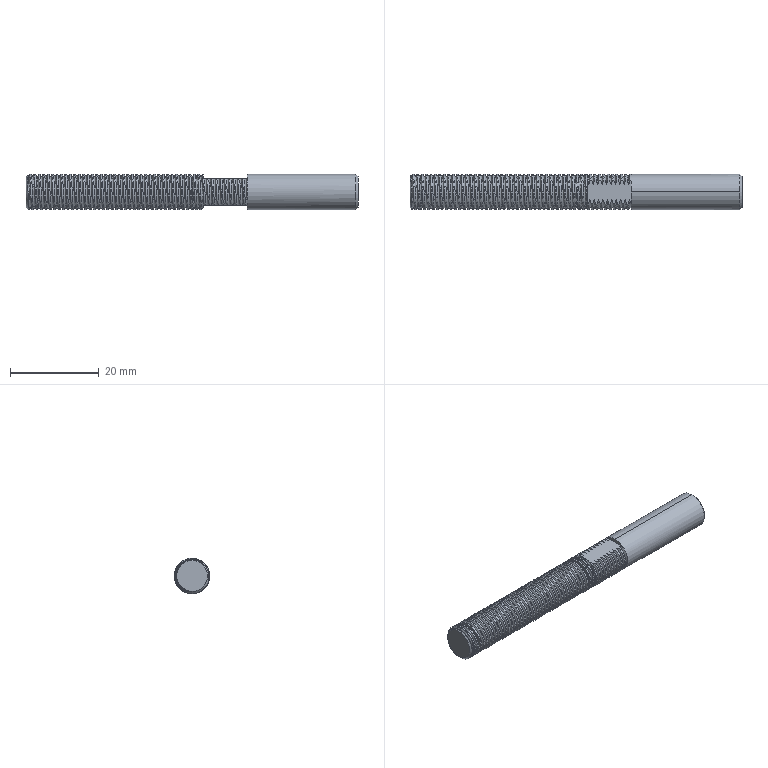Component | SolidWorks | NozzleConnectingPost-1 | 1 solid | 163 faces | volume 3190 mm3 | cylinder 103 | spline 42 | cone 9 | plane 9 | commonest cylinder face diameters 8 x101 5 x2